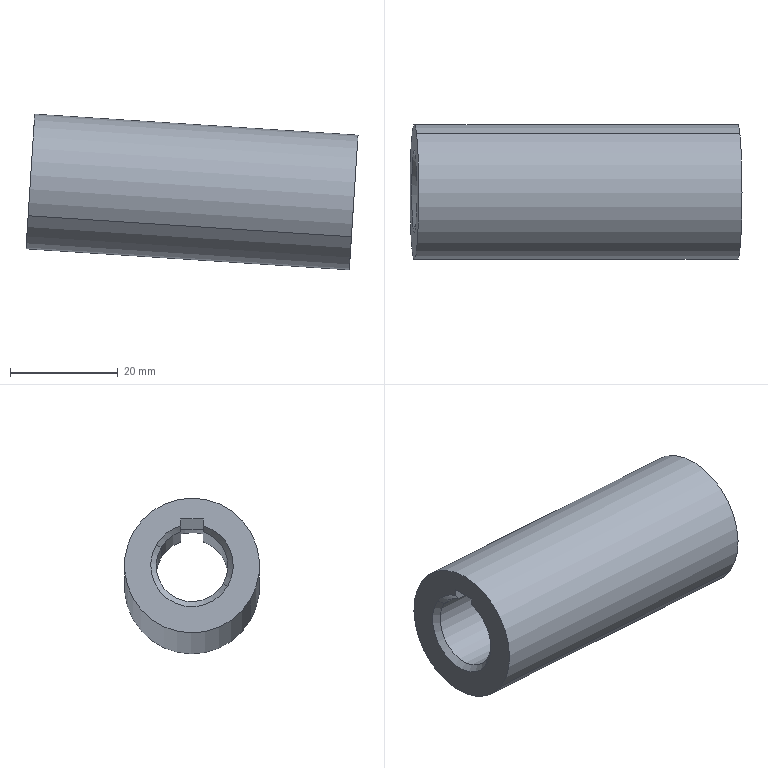Component | SolidWorks | Coupling-1 | 1 solid | 16 faces | box 61.49 x 25 x 28.83 mm | volume 15575 mm3 | cylinder 7 | plane 6 | cone 3 | commonest cylinder face diameters 13.3 x3 20 x2 25 x2
build123d program:
from build123d import *

# Parameters (mm, degrees)
SKETCH1_R               = 12.5
SKETCH1_R_2             = 10
BOSS_EXTRUDE1_DEPTH     = 30
BOSS_EXTRUDE2_START     = 30
SKETCH2_R               = 12.5
SKETCH2_R_2             = 6.65
BOSS_EXTRUDE2_DEPTH     = 30
CUT_EXTRUDE1_DEPTH      = 805.334
CUT_EXTRUDE1_DEPTH_BACK = 805.334
CHAMFER1_SIZE           = 1


with BuildPart() as part:
    # Sketch1 → Boss-Extrude1 (new body)
    with BuildSketch(Plane.XY):
        with Locations((300.503, -726)):
            Circle(SKETCH1_R)
        with Locations((300.503, -726)):
            Circle(SKETCH1_R_2, mode=Mode.SUBTRACT)
    extrude(amount=-BOSS_EXTRUDE1_DEPTH)

    # Sketch2 → Boss-Extrude2 (add)
    with BuildSketch(Plane.XY.offset(BOSS_EXTRUDE2_START)):
        with Locations((300.503, -726)):
            Circle(SKETCH2_R)
        with Locations((300.503, -726)):
            Circle(SKETCH2_R_2, mode=Mode.SUBTRACT)
    extrude(amount=-BOSS_EXTRUDE2_DEPTH)

    # Sketch3 → Cut-Extrude1 (cut, two sides: drawn at the far end of the back side and taken through both)
    with BuildSketch(Plane.XY.offset(30).offset(-CUT_EXTRUDE1_DEPTH_BACK)):
        Polygon((300.278, -721.485), (297.919, -717.495), (294.295, -719.638), (296.655, -723.628), align=None)
    extrude(amount=CUT_EXTRUDE1_DEPTH + CUT_EXTRUDE1_DEPTH_BACK, mode=Mode.SUBTRACT)

    # Chamfer1
    chamfer1_edges = [part.edges().sort_by_distance(p)[0] for p in [
        (303.887, -731.724, 30),
    ]]
    chamfer(chamfer1_edges, length=CHAMFER1_SIZE)


solid = part.part

# Placed as in the assembly
solid = solid.moved(Location((-68.732, -806.887, 494.123), (0, -86.288, -120.598)))
STEP:
#1=CARTESIAN_POINT('',(-5.819,-27.176,-10.9));
#2=VERTEX_POINT('',#1);
#3=CARTESIAN_POINT('',(-5.837,-27.627,-11.166));
#4=VERTEX_POINT('',#3);
#5=CARTESIAN_POINT('',(-5.828,-27.402,-11.033));
#6=DIRECTION('',(-0.9979,0.,0.06474));
#7=DIRECTION('',(-0.03295,-0.8608,-0.5079));
#8=AXIS2_PLACEMENT_3D('',#5,#6,#7);
#9=CIRCLE('',#8,0.2618);
#10=EDGE_CURVE('',#2,#4,#9,.T.);
#11=ORIENTED_EDGE('',*,*,#10,.F.);
#12=CARTESIAN_POINT('',(-5.857,-27.142,-10.877));
#13=VERTEX_POINT('',#12);
#14=CARTESIAN_POINT('',(-5.819,-27.176,-10.9));
#15=DIRECTION('',(-0.6823,0.6086,0.405));
#16=VECTOR('',#15,39.37);
#17=LINE('',#14,#16);
#18=EDGE_CURVE('',#2,#13,#17,.T.);
#19=ORIENTED_EDGE('',*,*,#18,.T.);
#20=CARTESIAN_POINT('',(-5.877,-27.661,-11.183));
#21=VERTEX_POINT('',#20);
#22=CARTESIAN_POINT('',(-5.867,-27.402,-11.03));
#23=DIRECTION('',(0.9979,-0.,-0.06474));
#24=DIRECTION('',(-0.03295,-0.8608,-0.5079));
#25=AXIS2_PLACEMENT_3D('',#22,#23,#24);
#26=CIRCLE('',#25,0.3012);
#27=EDGE_CURVE('',#21,#13,#26,.T.);
#28=ORIENTED_EDGE('',*,*,#27,.F.);
#29=CARTESIAN_POINT('',(-5.837,-27.627,-11.166));
#30=DIRECTION('',(-0.7289,-0.6086,-0.3134));
#31=VECTOR('',#30,39.37);
#32=LINE('',#29,#31);
#33=EDGE_CURVE('',#4,#21,#32,.T.);
#34=ORIENTED_EDGE('',*,*,#33,.F.);
#35=EDGE_LOOP('',(#11,#19,#28,#34));
#36=FACE_OUTER_BOUND('',#35,.T.);
#37=CARTESIAN_POINT('',(-5.828,-27.402,-11.033));
#38=DIRECTION('',(-0.9979,0.,0.06474));
#39=DIRECTION('',(-0.03295,-0.8608,-0.5079));
#40=AXIS2_PLACEMENT_3D('',#37,#38,#39);
#41=CONICAL_SURFACE('',#40,0.2618,0.7854);
#42=ADVANCED_FACE('',(#36),#41,.F.);
#43=CARTESIAN_POINT('',(-5.812,-27.484,-10.785));
#44=VERTEX_POINT('',#43);
#45=CARTESIAN_POINT('',(-5.828,-27.402,-11.033));
#46=DIRECTION('',(-0.9979,0.,0.06474));
#47=DIRECTION('',(-0.03295,-0.8608,-0.5079));
#48=AXIS2_PLACEMENT_3D('',#45,#46,#47);
#49=CIRCLE('',#48,0.2618);
#50=EDGE_CURVE('',#4,#44,#49,.T.);
#51=ORIENTED_EDGE('',*,*,#50,.F.);
#52=ORIENTED_EDGE('',*,*,#33,.T.);
#53=CARTESIAN_POINT('',(-5.849,-27.484,-10.741));
#54=VERTEX_POINT('',#53);
#55=CARTESIAN_POINT('',(-5.867,-27.402,-11.03));
#56=DIRECTION('',(0.9979,-0.,-0.06474));
#57=DIRECTION('',(-0.03295,-0.8608,-0.5079));
#58=AXIS2_PLACEMENT_3D('',#55,#56,#57);
#59=CIRCLE('',#58,0.3012);
#60=EDGE_CURVE('',#54,#21,#59,.T.);
#61=ORIENTED_EDGE('',*,*,#60,.F.);
#62=CARTESIAN_POINT('',(-5.812,-27.484,-10.785));
#63=CARTESIAN_POINT('',(-5.824,-27.484,-10.771));
#64=CARTESIAN_POINT('',(-5.836,-27.484,-10.756));
#65=CARTESIAN_POINT('',(-5.849,-27.484,-10.741));
#66=B_SPLINE_CURVE_WITH_KNOTS('',3,(#62,#63,#64,#65),.UNSPECIFIED.,.F.,.F.,(4,4),(0.,0.001448),.UNSPECIFIED.);
#67=EDGE_CURVE('',#44,#54,#66,.T.);
#68=ORIENTED_EDGE('',*,*,#67,.F.);
#69=EDGE_LOOP('',(#51,#52,#61,#68));
#70=FACE_OUTER_BOUND('',#69,.T.);
#71=CARTESIAN_POINT('',(-5.828,-27.402,-11.033));
#72=DIRECTION('',(-0.9979,0.,0.06474));
#73=DIRECTION('',(-0.03295,-0.8608,-0.5079));
#74=AXIS2_PLACEMENT_3D('',#71,#72,#73);
#75=CONICAL_SURFACE('',#74,0.2618,0.7854);
#76=ADVANCED_FACE('',(#70),#75,.F.);
#77=ORIENTED_EDGE('',*,*,#10,.T.);
#78=CARTESIAN_POINT('',(-4.697,-27.627,-11.24));
#79=VERTEX_POINT('',#78);
#80=CARTESIAN_POINT('',(-5.876,-27.627,-11.163));
#81=DIRECTION('',(0.9979,-0.,-0.06474));
#82=VECTOR('',#81,39.37);
#83=LINE('',#80,#82);
#84=EDGE_CURVE('',#4,#79,#83,.T.);
#85=ORIENTED_EDGE('',*,*,#84,.T.);
#86=CARTESIAN_POINT('',(-4.68,-27.176,-10.974));
#87=VERTEX_POINT('',#86);
#88=CARTESIAN_POINT('',(-4.689,-27.402,-11.107));
#89=DIRECTION('',(-0.9979,0.,0.06474));
#90=DIRECTION('',(-0.03295,-0.8608,-0.5079));
#91=AXIS2_PLACEMENT_3D('',#88,#89,#90);
#92=CIRCLE('',#91,0.2618);
#93=EDGE_CURVE('',#87,#79,#92,.T.);
#94=ORIENTED_EDGE('',*,*,#93,.F.);
#95=CARTESIAN_POINT('',(-5.859,-27.176,-10.897));
#96=DIRECTION('',(0.9979,-0.,-0.06474));
#97=VECTOR('',#96,39.37);
#98=LINE('',#95,#97);
#99=EDGE_CURVE('',#2,#87,#98,.T.);
#100=ORIENTED_EDGE('',*,*,#99,.F.);
#101=EDGE_LOOP('',(#77,#85,#94,#100));
#102=FACE_OUTER_BOUND('',#101,.T.);
#103=CARTESIAN_POINT('',(-5.867,-27.402,-11.03));
#104=DIRECTION('',(0.9979,-0.,-0.06474));
#105=DIRECTION('',(0.03295,0.8608,0.5079));
#106=AXIS2_PLACEMENT_3D('',#103,#104,#105);
#107=CYLINDRICAL_SURFACE('',#106,0.2618);
#108=ADVANCED_FACE('',(#102),#107,.F.);
#109=CARTESIAN_POINT('',(-5.812,-27.319,-10.785));
#110=VERTEX_POINT('',#109);
#111=CARTESIAN_POINT('',(-5.828,-27.402,-11.033));
#112=DIRECTION('',(-0.9979,0.,0.06474));
#113=DIRECTION('',(-0.03295,-0.8608,-0.5079));
#114=AXIS2_PLACEMENT_3D('',#111,#112,#113);
#115=CIRCLE('',#114,0.2618);
#116=EDGE_CURVE('',#110,#2,#115,.T.);
#117=ORIENTED_EDGE('',*,*,#116,.T.);
#118=ORIENTED_EDGE('',*,*,#99,.T.);
#119=CARTESIAN_POINT('',(-4.673,-27.319,-10.859));
#120=VERTEX_POINT('',#119);
#121=CARTESIAN_POINT('',(-4.689,-27.402,-11.107));
#122=DIRECTION('',(-0.9979,0.,0.06474));
#123=DIRECTION('',(-0.03295,-0.8608,-0.5079));
#124=AXIS2_PLACEMENT_3D('',#121,#122,#123);
#125=CIRCLE('',#124,0.2618);
#126=EDGE_CURVE('',#120,#87,#125,.T.);
#127=ORIENTED_EDGE('',*,*,#126,.F.);
#128=CARTESIAN_POINT('',(-5.851,-27.319,-10.783));
#129=DIRECTION('',(0.9979,-0.,-0.06474));
#130=VECTOR('',#129,39.37);
#131=LINE('',#128,#130);
#132=EDGE_CURVE('',#110,#120,#131,.T.);
#133=ORIENTED_EDGE('',*,*,#132,.F.);
#134=EDGE_LOOP('',(#117,#118,#127,#133));
#135=FACE_OUTER_BOUND('',#134,.T.);
#136=CARTESIAN_POINT('',(-5.867,-27.402,-11.03));
#137=DIRECTION('',(0.9979,-0.,-0.06474));
#138=DIRECTION('',(0.03295,0.8608,0.5079));
#139=AXIS2_PLACEMENT_3D('',#136,#137,#138);
#140=CYLINDRICAL_SURFACE('',#139,0.2618);
#141=ADVANCED_FACE('',(#135),#140,.F.);
#142=CARTESIAN_POINT('',(-3.497,-27.063,-10.983));
#143=VERTEX_POINT('',#142);
#144=CARTESIAN_POINT('',(-3.523,-27.74,-11.383));
#145=VERTEX_POINT('',#144);
#146=CARTESIAN_POINT('',(-3.51,-27.402,-11.183));
#147=DIRECTION('',(-0.9979,0.,0.06474));
#148=DIRECTION('',(-0.03295,-0.8608,-0.5079));
#149=AXIS2_PLACEMENT_3D('',#146,#147,#148);
#150=CIRCLE('',#149,0.3937);
#151=EDGE_CURVE('',#143,#145,#150,.T.);
#152=ORIENTED_EDGE('',*,*,#151,.F.);
#153=CARTESIAN_POINT('',(-4.676,-27.063,-10.907));
#154=VERTEX_POINT('',#153);
#155=CARTESIAN_POINT('',(-3.497,-27.063,-10.983));
#156=DIRECTION('',(-0.9979,0.,0.06474));
#157=VECTOR('',#156,39.37);
#158=LINE('',#155,#157);
#159=EDGE_CURVE('',#143,#154,#158,.T.);
#160=ORIENTED_EDGE('',*,*,#159,.T.);
#161=CARTESIAN_POINT('',(-4.702,-27.74,-11.307));
#162=VERTEX_POINT('',#161);
#163=CARTESIAN_POINT('',(-4.689,-27.402,-11.107));
#164=DIRECTION('',(-0.9979,0.,0.06474));
#165=DIRECTION('',(-0.03295,-0.8608,-0.5079));
#166=AXIS2_PLACEMENT_3D('',#163,#164,#165);
#167=CIRCLE('',#166,0.3937);
#168=EDGE_CURVE('',#154,#162,#167,.T.);
#169=ORIENTED_EDGE('',*,*,#168,.T.);
#170=CARTESIAN_POINT('',(-3.523,-27.74,-11.383));
#171=DIRECTION('',(-0.9979,0.,0.06474));
#172=VECTOR('',#171,39.37);
#173=LINE('',#170,#172);
#174=EDGE_CURVE('',#145,#162,#173,.T.);
#175=ORIENTED_EDGE('',*,*,#174,.F.);
#176=EDGE_LOOP('',(#152,#160,#169,#175));
#177=FACE_OUTER_BOUND('',#176,.T.);
#178=CARTESIAN_POINT('',(-3.51,-27.402,-11.183));
#179=DIRECTION('',(-0.9979,0.,0.06474));
#180=DIRECTION('',(-0.03295,-0.8608,-0.5079));
#181=AXIS2_PLACEMENT_3D('',#178,#179,#180);
#182=CYLINDRICAL_SURFACE('',#181,0.3937);
#183=ADVANCED_FACE('',(#177),#182,.F.);
#184=CARTESIAN_POINT('',(-3.526,-27.825,-11.433));
#185=VERTEX_POINT('',#184);
#186=CARTESIAN_POINT('',(-3.494,-26.978,-10.933));
#187=VERTEX_POINT('',#186);
#188=CARTESIAN_POINT('',(-3.51,-27.402,-11.183));
#189=DIRECTION('',(-0.9979,0.,0.06474));
#190=DIRECTION('',(-0.03295,-0.8608,-0.5079));
#191=AXIS2_PLACEMENT_3D('',#188,#189,#190);
#192=CIRCLE('',#191,0.4921);
#193=EDGE_CURVE('',#185,#187,#192,.T.);
#194=ORIENTED_EDGE('',*,*,#193,.T.);
#195=CARTESIAN_POINT('',(-5.851,-26.978,-10.78));
#196=VERTEX_POINT('',#195);
#197=CARTESIAN_POINT('',(-3.494,-26.978,-10.933));
#198=DIRECTION('',(-0.9979,0.,0.06474));
#199=VECTOR('',#198,39.37);
#200=LINE('',#197,#199);
#201=EDGE_CURVE('',#187,#196,#200,.T.);
#202=ORIENTED_EDGE('',*,*,#201,.T.);
#203=CARTESIAN_POINT('',(-5.884,-27.825,-11.28));
#204=VERTEX_POINT('',#203);
#205=CARTESIAN_POINT('',(-5.867,-27.402,-11.03));
#206=DIRECTION('',(-0.9979,0.,0.06474));
#207=DIRECTION('',(-0.03295,-0.8608,-0.5079));
#208=AXIS2_PLACEMENT_3D('',#205,#206,#207);
#209=CIRCLE('',#208,0.4921);
#210=EDGE_CURVE('',#204,#196,#209,.T.);
#211=ORIENTED_EDGE('',*,*,#210,.F.);
#212=CARTESIAN_POINT('',(-3.526,-27.825,-11.433));
#213=DIRECTION('',(-0.9979,0.,0.06474));
#214=VECTOR('',#213,39.37);
#215=LINE('',#212,#214);
#216=EDGE_CURVE('',#185,#204,#215,.T.);
#217=ORIENTED_EDGE('',*,*,#216,.F.);
#218=EDGE_LOOP('',(#194,#202,#211,#217));
#219=FACE_OUTER_BOUND('',#218,.T.);
#220=CARTESIAN_POINT('',(-3.51,-27.402,-11.183));
#221=DIRECTION('',(-0.9979,0.,0.06474));
#222=DIRECTION('',(-0.03295,-0.8608,-0.5079));
#223=AXIS2_PLACEMENT_3D('',#220,#221,#222);
#224=CYLINDRICAL_SURFACE('',#223,0.4921);
#225=ADVANCED_FACE('',(#219),#224,.T.);
#226=ORIENTED_EDGE('',*,*,#201,.F.);
#227=CARTESIAN_POINT('',(-3.51,-27.402,-11.183));
#228=DIRECTION('',(-0.9979,0.,0.06474));
#229=DIRECTION('',(-0.03295,-0.8608,-0.5079));
#230=AXIS2_PLACEMENT_3D('',#227,#228,#229);
#231=CIRCLE('',#230,0.4921);
#232=EDGE_CURVE('',#187,#185,#231,.T.);
#233=ORIENTED_EDGE('',*,*,#232,.T.);
#234=ORIENTED_EDGE('',*,*,#216,.T.);
#235=CARTESIAN_POINT('',(-5.867,-27.402,-11.03));
#236=DIRECTION('',(-0.9979,0.,0.06474));
#237=DIRECTION('',(-0.03295,-0.8608,-0.5079));
#238=AXIS2_PLACEMENT_3D('',#235,#236,#237);
#239=CIRCLE('',#238,0.4921);
#240=EDGE_CURVE('',#196,#204,#239,.T.);
#241=ORIENTED_EDGE('',*,*,#240,.F.);
#242=EDGE_LOOP('',(#226,#233,#234,#241));
#243=FACE_OUTER_BOUND('',#242,.T.);
#244=CARTESIAN_POINT('',(-3.51,-27.402,-11.183));
#245=DIRECTION('',(-0.9979,0.,0.06474));
#246=DIRECTION('',(-0.03295,-0.8608,-0.5079));
#247=AXIS2_PLACEMENT_3D('',#244,#245,#246);
#248=CYLINDRICAL_SURFACE('',#247,0.4921);
#249=ADVANCED_FACE('',(#243),#248,.T.);
#250=CARTESIAN_POINT('',(-3.51,-27.402,-11.183));
#251=DIRECTION('',(-0.9979,0.,0.06474));
#252=DIRECTION('',(-0.03295,-0.8608,-0.5079));
#253=AXIS2_PLACEMENT_3D('',#250,#251,#252);
#254=CIRCLE('',#253,0.3937);
#255=EDGE_CURVE('',#145,#143,#254,.T.);
#256=ORIENTED_EDGE('',*,*,#255,.T.);
#257=ORIENTED_EDGE('',*,*,#151,.T.);
#258=EDGE_LOOP('',(#256,#257));
#259=FACE_BOUND('',#258,.T.);
#260=ORIENTED_EDGE('',*,*,#193,.F.);
#261=ORIENTED_EDGE('',*,*,#232,.F.);
#262=EDGE_LOOP('',(#260,#261));
#263=FACE_OUTER_BOUND('',#262,.T.);
#264=CARTESIAN_POINT('',(-3.51,-27.402,-11.183));
#265=DIRECTION('',(-0.9979,0.,0.06474));
#266=DIRECTION('',(-0.03295,-0.8608,-0.5079));
#267=AXIS2_PLACEMENT_3D('',#264,#265,#266);
#268=PLANE('',#267);
#269=ADVANCED_FACE('',(#259,#263),#268,.F.);
#270=ORIENTED_EDGE('',*,*,#159,.F.);
#271=ORIENTED_EDGE('',*,*,#255,.F.);
#272=ORIENTED_EDGE('',*,*,#174,.T.);
#273=CARTESIAN_POINT('',(-4.689,-27.402,-11.107));
#274=DIRECTION('',(-0.9979,0.,0.06474));
#275=DIRECTION('',(-0.03295,-0.8608,-0.5079));
#276=AXIS2_PLACEMENT_3D('',#273,#274,#275);
#277=CIRCLE('',#276,0.3937);
#278=EDGE_CURVE('',#162,#154,#277,.T.);
#279=ORIENTED_EDGE('',*,*,#278,.T.);
#280=EDGE_LOOP('',(#270,#271,#272,#279));
#281=FACE_OUTER_BOUND('',#280,.T.);
#282=CARTESIAN_POINT('',(-3.51,-27.402,-11.183));
#283=DIRECTION('',(-0.9979,0.,0.06474));
#284=DIRECTION('',(-0.03295,-0.8608,-0.5079));
#285=AXIS2_PLACEMENT_3D('',#282,#283,#284);
#286=CYLINDRICAL_SURFACE('',#285,0.3937);
#287=ADVANCED_FACE('',(#281),#286,.F.);
#288=CARTESIAN_POINT('',(-4.667,-27.484,-10.768));
#289=VERTEX_POINT('',#288);
#290=CARTESIAN_POINT('',(-4.667,-27.319,-10.768));
#291=VERTEX_POINT('',#290);
#292=CARTESIAN_POINT('',(-4.667,-27.402,-10.768));
#293=DIRECTION('',(-0.,1.,-0.));
#294=VECTOR('',#293,39.37);
#295=LINE('',#292,#294);
#296=EDGE_CURVE('',#289,#291,#295,.T.);
#297=ORIENTED_EDGE('',*,*,#296,.T.);
#298=CARTESIAN_POINT('',(-4.689,-27.319,-11.107));
#299=DIRECTION('',(-0.06474,-0.,-0.9979));
#300=VECTOR('',#299,39.37);
#301=LINE('',#298,#300);
#302=EDGE_CURVE('',#291,#120,#301,.T.);
#303=ORIENTED_EDGE('',*,*,#302,.T.);
#304=ORIENTED_EDGE('',*,*,#126,.T.);
#305=ORIENTED_EDGE('',*,*,#93,.T.);
#306=CARTESIAN_POINT('',(-4.673,-27.484,-10.859));
#307=VERTEX_POINT('',#306);
#308=CARTESIAN_POINT('',(-4.689,-27.402,-11.107));
#309=DIRECTION('',(-0.9979,0.,0.06474));
#310=DIRECTION('',(-0.03295,-0.8608,-0.5079));
#311=AXIS2_PLACEMENT_3D('',#308,#309,#310);
#312=CIRCLE('',#311,0.2618);
#313=EDGE_CURVE('',#79,#307,#312,.T.);
#314=ORIENTED_EDGE('',*,*,#313,.T.);
#315=CARTESIAN_POINT('',(-4.689,-27.484,-11.107));
#316=DIRECTION('',(0.06474,-0.,0.9979));
#317=VECTOR('',#316,39.37);
#318=LINE('',#315,#317);
#319=EDGE_CURVE('',#307,#289,#318,.T.);
#320=ORIENTED_EDGE('',*,*,#319,.T.);
#321=EDGE_LOOP('',(#297,#303,#304,#305,#314,#320));
#322=FACE_BOUND('',#321,.T.);
#323=ORIENTED_EDGE('',*,*,#278,.F.);
#324=ORIENTED_EDGE('',*,*,#168,.F.);
#325=EDGE_LOOP('',(#323,#324));
#326=FACE_OUTER_BOUND('',#325,.T.);
#327=CARTESIAN_POINT('',(-4.689,-27.402,-11.107));
#328=DIRECTION('',(-0.9979,0.,0.06474));
#329=DIRECTION('',(-0.03295,-0.8608,-0.5079));
#330=AXIS2_PLACEMENT_3D('',#327,#328,#329);
#331=PLANE('',#330);
#332=ADVANCED_FACE('',(#322,#326),#331,.F.);
#333=CARTESIAN_POINT('',(-5.845,-27.484,-10.691));
#334=VERTEX_POINT('',#333);
#335=CARTESIAN_POINT('',(-5.867,-27.484,-11.03));
#336=DIRECTION('',(0.06474,-0.,0.9979));
#337=VECTOR('',#336,39.37);
#338=LINE('',#335,#337);
#339=EDGE_CURVE('',#54,#334,#338,.T.);
#340=ORIENTED_EDGE('',*,*,#339,.F.);
#341=ORIENTED_EDGE('',*,*,#60,.T.);
#342=ORIENTED_EDGE('',*,*,#27,.T.);
#343=CARTESIAN_POINT('',(-5.849,-27.319,-10.741));
#344=VERTEX_POINT('',#343);
#345=CARTESIAN_POINT('',(-5.867,-27.402,-11.03));
#346=DIRECTION('',(0.9979,-0.,-0.06474));
#347=DIRECTION('',(-0.03295,-0.8608,-0.5079));
#348=AXIS2_PLACEMENT_3D('',#345,#346,#347);
#349=CIRCLE('',#348,0.3012);
#350=EDGE_CURVE('',#13,#344,#349,.T.);
#351=ORIENTED_EDGE('',*,*,#350,.T.);
#352=CARTESIAN_POINT('',(-5.845,-27.319,-10.691));
#353=VERTEX_POINT('',#352);
#354=CARTESIAN_POINT('',(-5.867,-27.319,-11.03));
#355=DIRECTION('',(-0.06474,-0.,-0.9979));
#356=VECTOR('',#355,39.37);
#357=LINE('',#354,#356);
#358=EDGE_CURVE('',#353,#344,#357,.T.);
#359=ORIENTED_EDGE('',*,*,#358,.F.);
#360=CARTESIAN_POINT('',(-5.845,-27.402,-10.691));
#361=DIRECTION('',(-0.,1.,-0.));
#362=VECTOR('',#361,39.37);
#363=LINE('',#360,#362);
#364=EDGE_CURVE('',#334,#353,#363,.T.);
#365=ORIENTED_EDGE('',*,*,#364,.F.);
#366=EDGE_LOOP('',(#340,#341,#342,#351,#359,#365));
#367=FACE_BOUND('',#366,.T.);
#368=ORIENTED_EDGE('',*,*,#210,.T.);
#369=ORIENTED_EDGE('',*,*,#240,.T.);
#370=EDGE_LOOP('',(#368,#369));
#371=FACE_OUTER_BOUND('',#370,.T.);
#372=CARTESIAN_POINT('',(-5.867,-27.402,-11.03));
#373=DIRECTION('',(-0.9979,0.,0.06474));
#374=DIRECTION('',(-0.03295,-0.8608,-0.5079));
#375=AXIS2_PLACEMENT_3D('',#372,#373,#374);
#376=PLANE('',#375);
#377=ADVANCED_FACE('',(#367,#371),#376,.T.);
#378=ORIENTED_EDGE('',*,*,#84,.F.);
#379=ORIENTED_EDGE('',*,*,#50,.T.);
#380=CARTESIAN_POINT('',(-5.851,-27.484,-10.783));
#381=DIRECTION('',(-0.9979,0.,0.06474));
#382=VECTOR('',#381,39.37);
#383=LINE('',#380,#382);
#384=EDGE_CURVE('',#307,#44,#383,.T.);
#385=ORIENTED_EDGE('',*,*,#384,.F.);
#386=ORIENTED_EDGE('',*,*,#313,.F.);
#387=EDGE_LOOP('',(#378,#379,#385,#386));
#388=FACE_OUTER_BOUND('',#387,.T.);
#389=CARTESIAN_POINT('',(-5.867,-27.402,-11.03));
#390=DIRECTION('',(0.9979,-0.,-0.06474));
#391=DIRECTION('',(0.03295,0.8608,0.5079));
#392=AXIS2_PLACEMENT_3D('',#389,#390,#391);
#393=CYLINDRICAL_SURFACE('',#392,0.2618);
#394=ADVANCED_FACE('',(#388),#393,.F.);
#395=CARTESIAN_POINT('',(-3.488,-27.484,-10.844));
#396=DIRECTION('',(-0.9979,0.,0.06474));
#397=VECTOR('',#396,39.37);
#398=LINE('',#395,#397);
#399=EDGE_CURVE('',#289,#334,#398,.T.);
#400=ORIENTED_EDGE('',*,*,#399,.T.);
#401=ORIENTED_EDGE('',*,*,#364,.T.);
#402=CARTESIAN_POINT('',(-3.488,-27.319,-10.844));
#403=DIRECTION('',(-0.9979,0.,0.06474));
#404=VECTOR('',#403,39.37);
#405=LINE('',#402,#404);
#406=EDGE_CURVE('',#291,#353,#405,.T.);
#407=ORIENTED_EDGE('',*,*,#406,.F.);
#408=ORIENTED_EDGE('',*,*,#296,.F.);
#409=EDGE_LOOP('',(#400,#401,#407,#408));
#410=FACE_OUTER_BOUND('',#409,.T.);
#411=CARTESIAN_POINT('',(-3.488,-27.484,-10.844));
#412=DIRECTION('',(0.06474,0.,0.9979));
#413=DIRECTION('',(-0.,1.,-0.));
#414=AXIS2_PLACEMENT_3D('',#411,#412,#413);
#415=PLANE('',#414);
#416=ADVANCED_FACE('',(#410),#415,.F.);
#417=ORIENTED_EDGE('',*,*,#358,.T.);
#418=CARTESIAN_POINT('',(-5.849,-27.319,-10.741));
#419=CARTESIAN_POINT('',(-5.836,-27.319,-10.756));
#420=CARTESIAN_POINT('',(-5.824,-27.319,-10.771));
#421=CARTESIAN_POINT('',(-5.812,-27.319,-10.785));
#422=B_SPLINE_CURVE_WITH_KNOTS('',3,(#418,#419,#420,#421),.UNSPECIFIED.,.F.,.F.,(4,4),(0.,0.001448),.UNSPECIFIED.);
#423=EDGE_CURVE('',#344,#110,#422,.T.);
#424=ORIENTED_EDGE('',*,*,#423,.T.);
#425=ORIENTED_EDGE('',*,*,#132,.T.);
#426=ORIENTED_EDGE('',*,*,#302,.F.);
#427=ORIENTED_EDGE('',*,*,#406,.T.);
#428=EDGE_LOOP('',(#417,#424,#425,#426,#427));
#429=FACE_OUTER_BOUND('',#428,.T.);
#430=CARTESIAN_POINT('',(-3.5,-27.319,-11.026));
#431=DIRECTION('',(0.,1.,-0.));
#432=DIRECTION('',(-0.06474,-0.,-0.9979));
#433=AXIS2_PLACEMENT_3D('',#430,#431,#432);
#434=PLANE('',#433);
#435=ADVANCED_FACE('',(#429),#434,.F.);
#436=ORIENTED_EDGE('',*,*,#384,.T.);
#437=ORIENTED_EDGE('',*,*,#67,.T.);
#438=ORIENTED_EDGE('',*,*,#339,.T.);
#439=ORIENTED_EDGE('',*,*,#399,.F.);
#440=ORIENTED_EDGE('',*,*,#319,.F.);
#441=EDGE_LOOP('',(#436,#437,#438,#439,#440));
#442=FACE_OUTER_BOUND('',#441,.T.);
#443=CARTESIAN_POINT('',(-3.5,-27.484,-11.026));
#444=DIRECTION('',(-0.,-1.,-0.));
#445=DIRECTION('',(0.06474,-0.,0.9979));
#446=AXIS2_PLACEMENT_3D('',#443,#444,#445);
#447=PLANE('',#446);
#448=ADVANCED_FACE('',(#442),#447,.F.);
#449=ORIENTED_EDGE('',*,*,#18,.F.);
#450=ORIENTED_EDGE('',*,*,#116,.F.);
#451=ORIENTED_EDGE('',*,*,#423,.F.);
#452=ORIENTED_EDGE('',*,*,#350,.F.);
#453=EDGE_LOOP('',(#449,#450,#451,#452));
#454=FACE_OUTER_BOUND('',#453,.T.);
#455=CARTESIAN_POINT('',(-5.828,-27.402,-11.033));
#456=DIRECTION('',(-0.9979,0.,0.06474));
#457=DIRECTION('',(-0.03295,-0.8608,-0.5079));
#458=AXIS2_PLACEMENT_3D('',#455,#456,#457);
#459=CONICAL_SURFACE('',#458,0.2618,0.7854);
#460=ADVANCED_FACE('',(#454),#459,.F.);
#461=CLOSED_SHELL('',(#42,#76,#108,#141,#183,#225,#249,#269,#287,#332,#377,#394,#416,#435,#448,#460));
#462=MANIFOLD_SOLID_BREP('',#461);
#463=CARTESIAN_POINT('',(0.,0.,0.));
#464=DIRECTION('',(0.,0.,1.));
#465=DIRECTION('',(1.,0.,0.));
#466=AXIS2_PLACEMENT_3D('',#463,#464,#465);
#467=(LENGTH_UNIT()NAMED_UNIT(*)SI_UNIT($,.METRE.));
#468=LENGTH_MEASURE_WITH_UNIT(LENGTH_MEASURE(0.0254),#467);
#469=DIMENSIONAL_EXPONENTS(1.,0.,0.,0.,0.,0.,0.);
#470=(CONVERSION_BASED_UNIT('',#468)LENGTH_UNIT()NAMED_UNIT(#469));
#471=UNCERTAINTY_MEASURE_WITH_UNIT(LENGTH_MEASURE(0.00001),#470,'','');
#472=(NAMED_UNIT(*)PLANE_ANGLE_UNIT()SI_UNIT($,.RADIAN.));
#473=(NAMED_UNIT(*)SI_UNIT($,.STERADIAN.)SOLID_ANGLE_UNIT());
#474=(GEOMETRIC_REPRESENTATION_CONTEXT(3)GLOBAL_UNCERTAINTY_ASSIGNED_CONTEXT((#471))GLOBAL_UNIT_ASSIGNED_CONTEXT((#470,#472,#473))REPRESENTATION_CONTEXT('',''));
#475=ADVANCED_BREP_SHAPE_REPRESENTATION('',(#462,#466),#474);
#476=COLOUR_RGB('',0.7922,0.8196,0.9333);
#477=FILL_AREA_STYLE_COLOUR('',#476);
#478=FILL_AREA_STYLE('',(#477));
#479=SURFACE_STYLE_FILL_AREA(#478);
#480=SURFACE_SIDE_STYLE('',(#479));
#481=SURFACE_STYLE_USAGE(.BOTH.,#480);
#482=PRESENTATION_STYLE_ASSIGNMENT((#481));
#483=STYLED_ITEM('',(#482),#462);
#484=PRESENTATION_LAYER_ASSIGNMENT('','',(#483));
#485=(LENGTH_UNIT()NAMED_UNIT(*)SI_UNIT($,.METRE.));
#486=LENGTH_MEASURE_WITH_UNIT(LENGTH_MEASURE(0.0254),#485);
#487=DIMENSIONAL_EXPONENTS(1.,0.,0.,0.,0.,0.,0.);
#488=(CONVERSION_BASED_UNIT('',#486)LENGTH_UNIT()NAMED_UNIT(#487));
#489=UNCERTAINTY_MEASURE_WITH_UNIT(LENGTH_MEASURE(0.00001),#488,'','');
#490=(NAMED_UNIT(*)PLANE_ANGLE_UNIT()SI_UNIT($,.RADIAN.));
#491=(NAMED_UNIT(*)SI_UNIT($,.STERADIAN.)SOLID_ANGLE_UNIT());
#492=(GEOMETRIC_REPRESENTATION_CONTEXT(3)GLOBAL_UNCERTAINTY_ASSIGNED_CONTEXT((#489))GLOBAL_UNIT_ASSIGNED_CONTEXT((#488,#490,#491))REPRESENTATION_CONTEXT('',''));
#493=MECHANICAL_DESIGN_GEOMETRIC_PRESENTATION_REPRESENTATION('',(#483),#492);